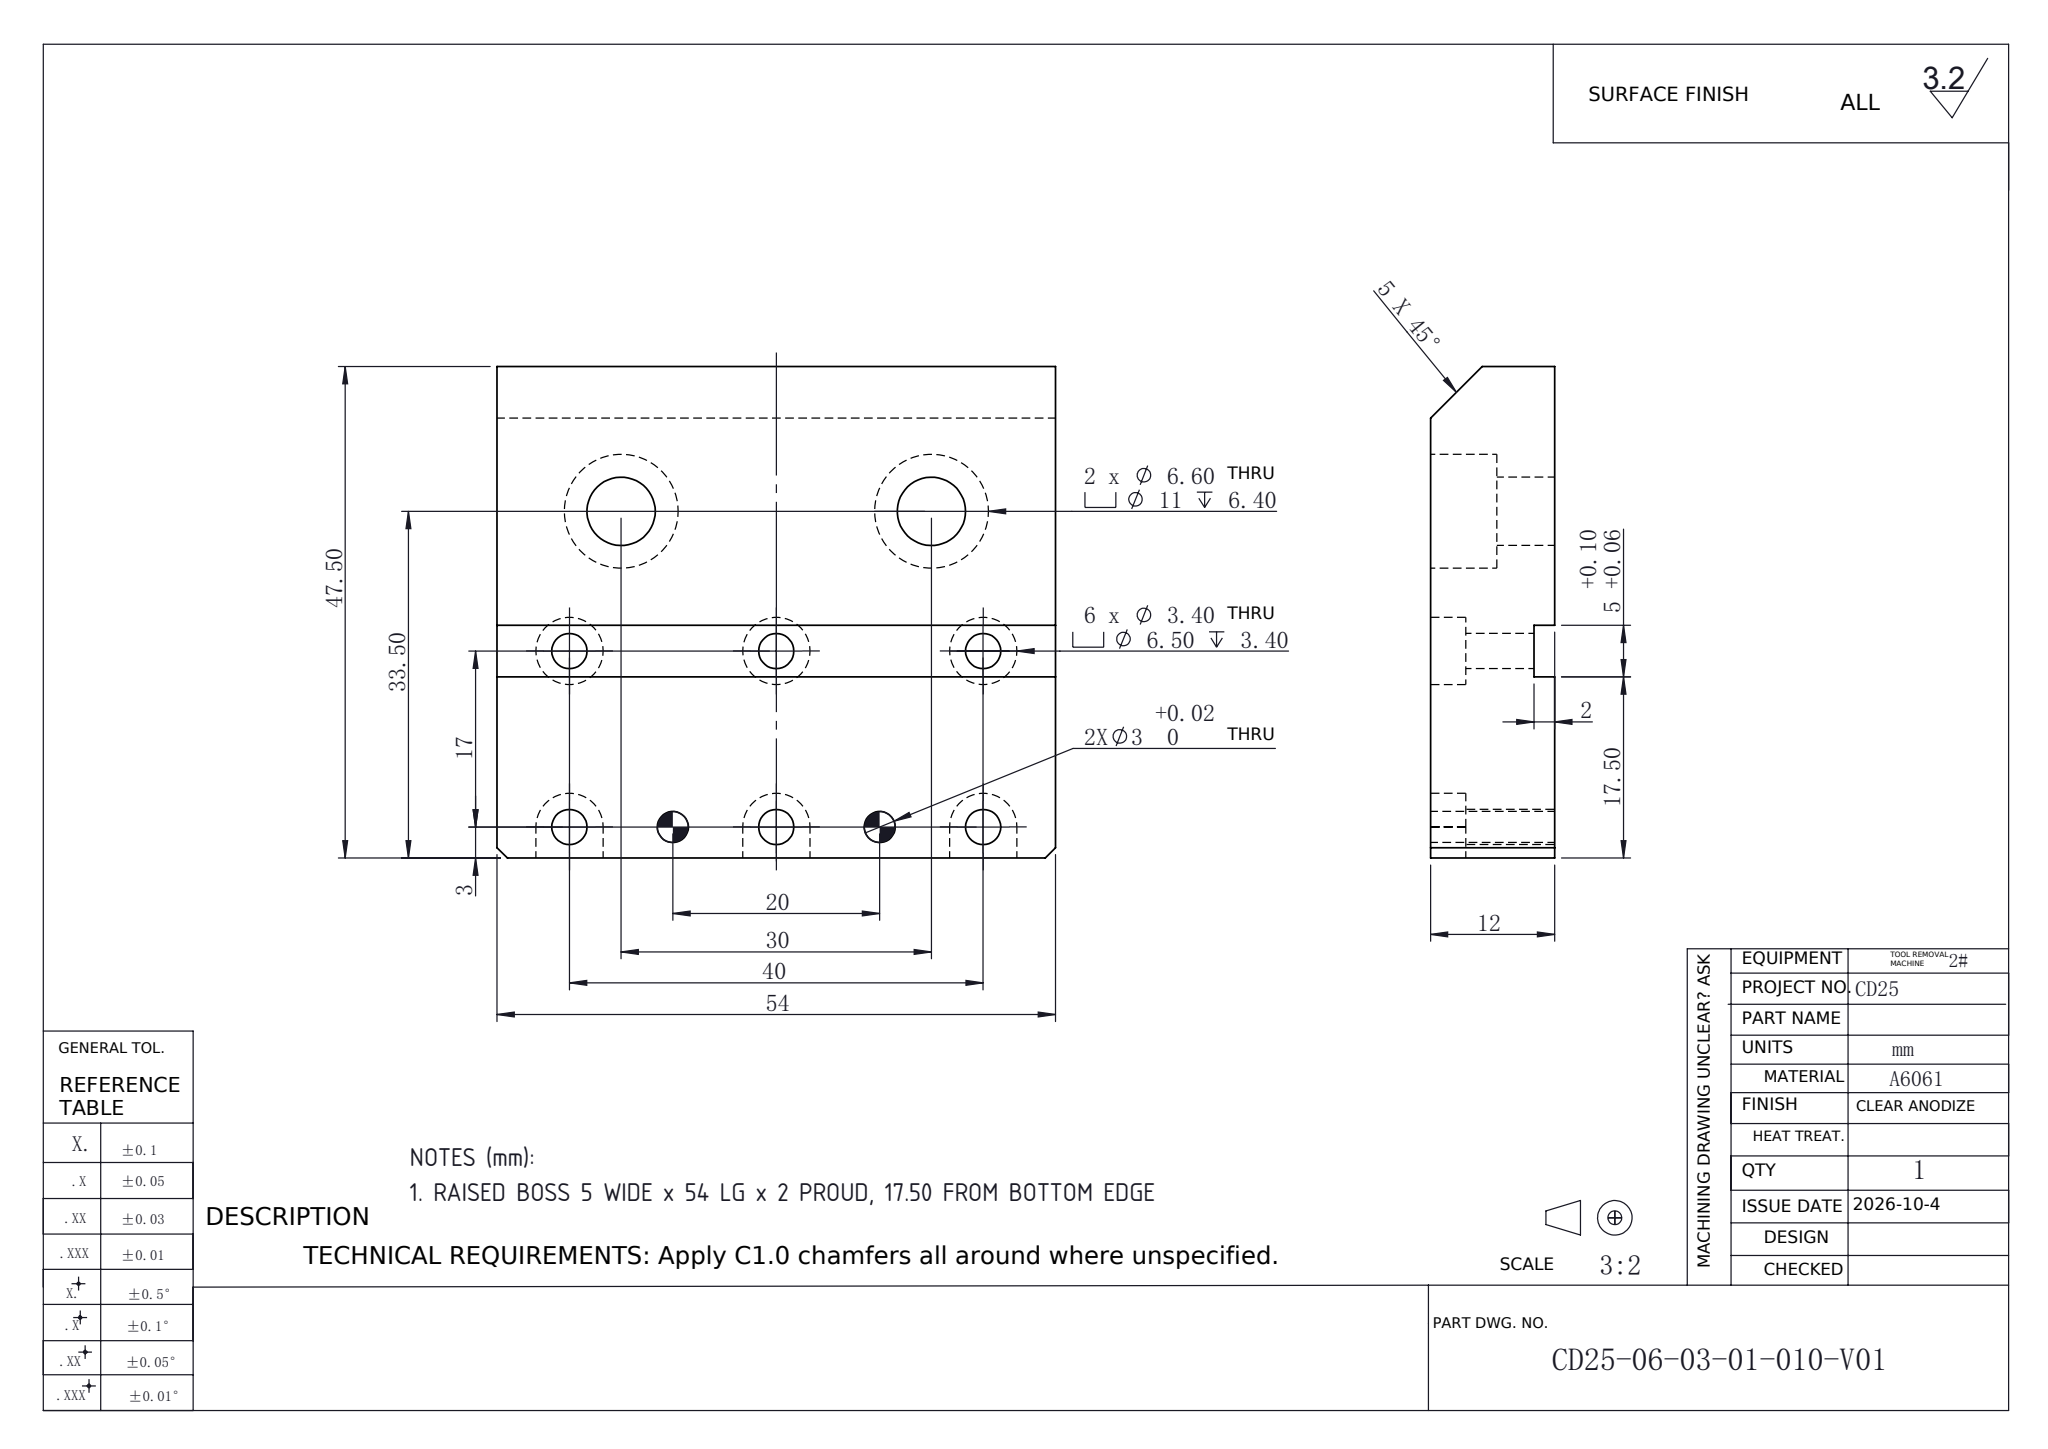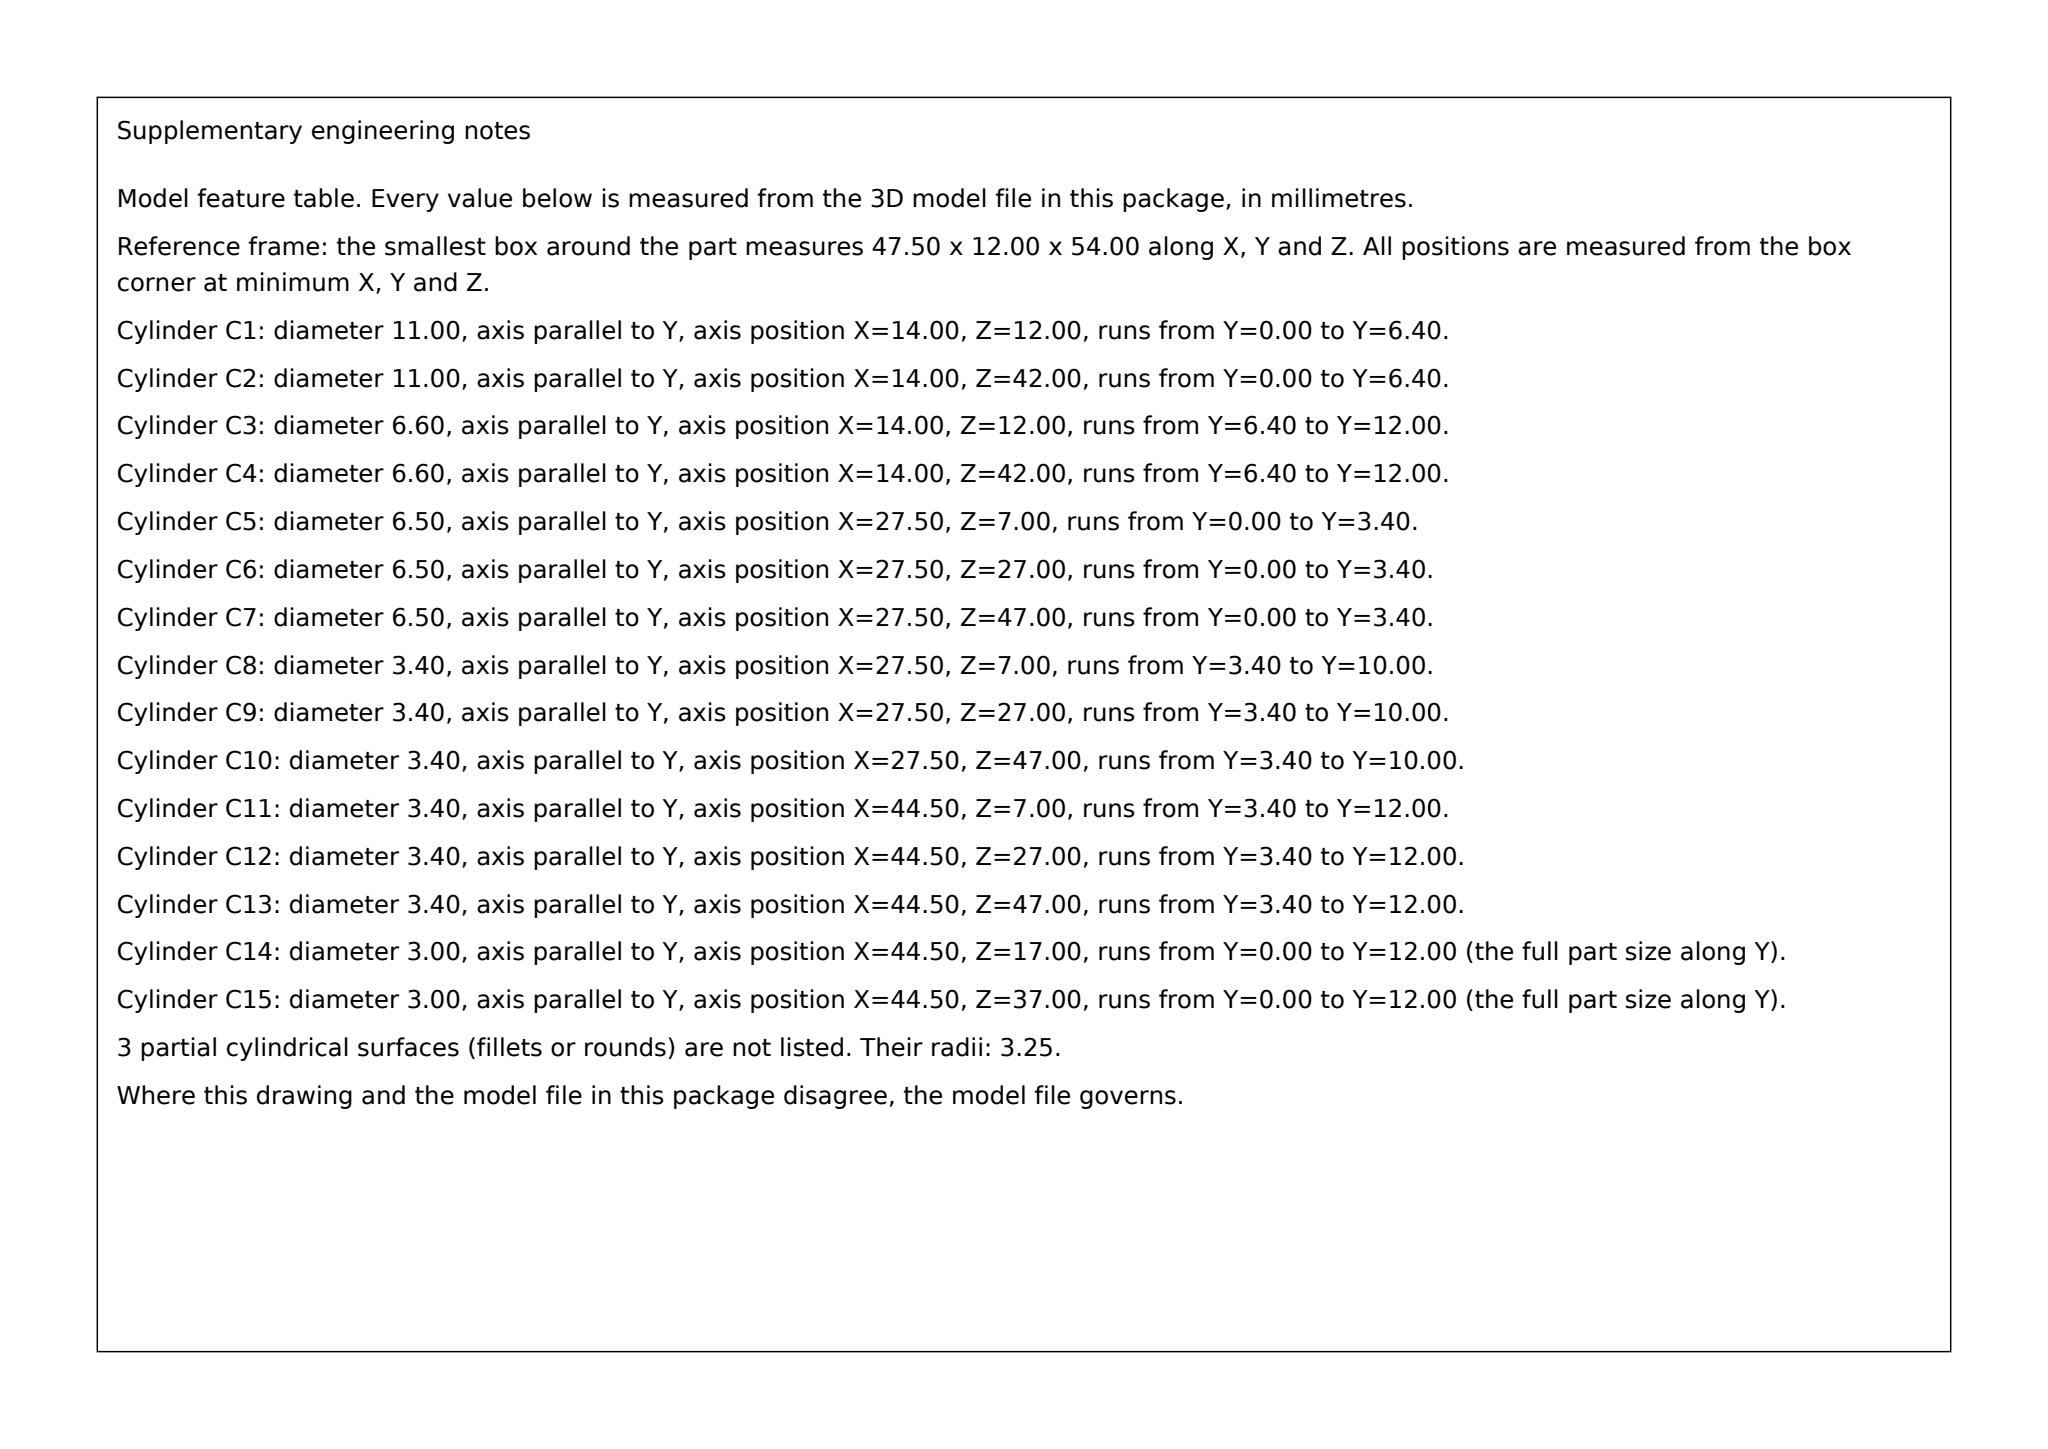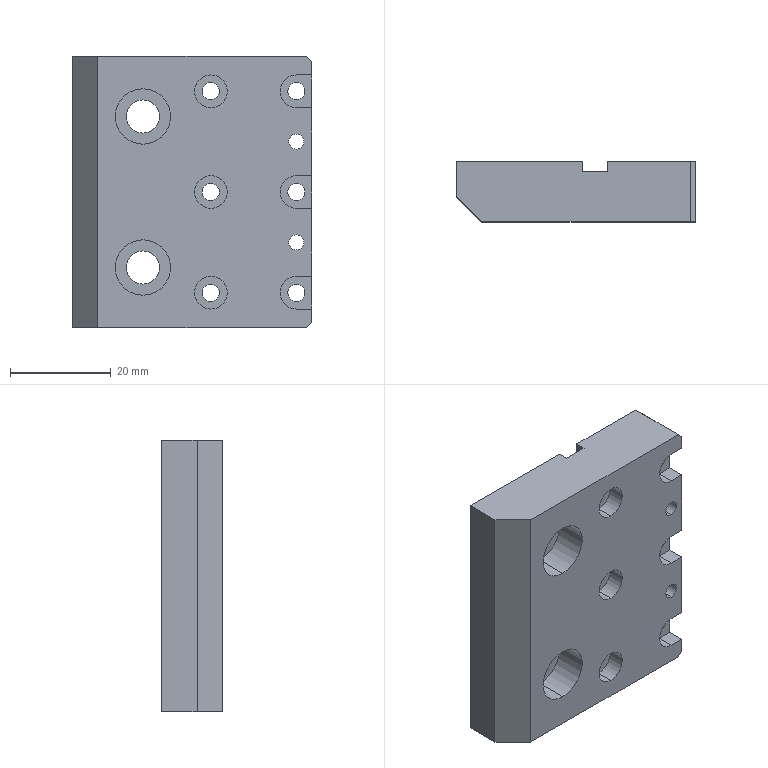Part | SolidWorks | mm | 1 solid | 60 faces | box 47.5 x 12 x 54 mm | volume 26663 mm3 | cylinder 33 | plane 27 | commonest cylinder face diameters 3.4 x12 6.5 x9 3 x4 11 x4 6.6 x4
Drawing notes:
RAISED BOSS 5 WIDE x 54 LG x 2 PROUD, 17.50 FROM BOTTOM EDGE | from the solid: x-planes at 25.0 & 30.0 (5 wide) on 47.5 height => 17.5 to 22.5 from bottom edge; boss spans full z=0 to 54; y-planes 10.0 to 12.0 give 2 thk
build123d program:
from build123d import *

# Parameters (mm, degrees)
SKETCH1_W                                       = 47.5
SKETCH1_H                                       = 54
BOSS_EXTRUDE1_DEPTH                             = 6
M6_HEX_SOCKET_HEAD_CAP_SCREW_CBORE1_D           = 6.6
M6_HEX_SOCKET_HEAD_CAP_SCREW_CBORE1_CBORE_D     = 11
M6_HEX_SOCKET_HEAD_CAP_SCREW_CBORE1_CBORE_DEPTH = 6.4
M3_HEX_SOCKET_HEAD_CAP_SCREW_CBORE1_D           = 3.4
M3_HEX_SOCKET_HEAD_CAP_SCREW_CBORE1_CBORE_D     = 6.5
M3_HEX_SOCKET_HEAD_CAP_SCREW_CBORE1_CBORE_DEPTH = 3.4
F_3_0MM_DOWEL_PIN_HOLE1_D                       = 3
CUT_EXTRUDE1_DEPTH                              = 3.4
CHAMFER1_SIZE                                   = 1
SKETCH10_W                                      = 5
SKETCH10_H                                      = 2
CUT_EXTRUDE2_DEPTH                              = 60.296
CHAMFER2_SIZE                                   = 5


with BuildPart() as part:
    # Sketch1 → Boss-Extrude1 (new, symmetric)
    with BuildSketch(Plane(origin=(0, 0, 0), x_dir=(1, 0, 0), z_dir=(0, 1, 0))):
        Rectangle(SKETCH1_W, SKETCH1_H)
    extrude(amount=BOSS_EXTRUDE1_DEPTH, both=True)

    # M6 Hex Socket Head Cap Screw CBORE1 (through all)
    with Locations(Plane(origin=(0, -6, 0), x_dir=(-1, 0, 0), z_dir=(0, -1, 0))):
        with Locations((9.75, 15), (9.75, -15)):
            CounterBoreHole(M6_HEX_SOCKET_HEAD_CAP_SCREW_CBORE1_D / 2, M6_HEX_SOCKET_HEAD_CAP_SCREW_CBORE1_CBORE_D / 2, M6_HEX_SOCKET_HEAD_CAP_SCREW_CBORE1_CBORE_DEPTH)

    # M3 Hex Socket Head Cap Screw CBORE1 (through all)
    with Locations(Plane(origin=(0, -6, 0), x_dir=(-1, 0, 0), z_dir=(0, -1, 0))):
        with Locations((-20.75, -20), (-20.75, 0), (-20.75, 20), (-3.75, 20), (-3.75, 0), (-3.75, -20)):
            CounterBoreHole(M3_HEX_SOCKET_HEAD_CAP_SCREW_CBORE1_D / 2, M3_HEX_SOCKET_HEAD_CAP_SCREW_CBORE1_CBORE_D / 2, M3_HEX_SOCKET_HEAD_CAP_SCREW_CBORE1_CBORE_DEPTH)

    # 3.0mm Dowel Pin Hole1 (through all)
    with Locations(Plane(origin=(0, -6, 0), x_dir=(-1, 0, 0), z_dir=(0, -1, 0))):
        with Locations((-20.75, 10), (-20.75, -10)):
            Hole(F_3_0MM_DOWEL_PIN_HOLE1_D / 2)

    # Sketch9 → Cut-Extrude1 (cut)
    with BuildSketch(Plane.XZ.offset(6)):
        with BuildLine():
            Line((20.75, 23.25), (23.75, 23.25))
            ThreePointArc((23.75, 23.25), (27, 20), (23.75, 16.75))
            Line((23.75, 16.75), (20.75, 16.75))
            ThreePointArc((20.75, 16.75), (17.5, 20), (20.75, 23.25))
        make_face()
        with BuildLine():
            Line((20.75, -23.25), (23.75, -23.25))
            ThreePointArc((23.75, -23.25), (27, -20), (23.75, -16.75))
            Line((23.75, -16.75), (20.75, -16.75))
            ThreePointArc((20.75, -16.75), (17.5, -20), (20.75, -23.25))
        make_face()
        with BuildLine():
            Line((20.75, 3.25), (23.75, 3.25))
            ThreePointArc((23.75, 3.25), (27, 0), (23.75, -3.25))
            Line((23.75, -3.25), (20.75, -3.25))
            ThreePointArc((20.75, -3.25), (17.5, 0), (20.75, 3.25))
        make_face()
    extrude(amount=-CUT_EXTRUDE1_DEPTH, mode=Mode.SUBTRACT)

    # Chamfer1
    chamfer1_edges = [part.edges().sort_by_distance(p)[0] for p in [
        (23.75, 0, 27),
        (23.75, 0, -27),
    ]]
    chamfer(chamfer1_edges, length=CHAMFER1_SIZE)

    # Sketch10 → Cut-Extrude2 (cut, through all)
    with BuildSketch(Plane(origin=(0, 0, -27), x_dir=(-1, 0, 0), z_dir=(0, 0, -1))):
        with Locations((-3.75, 5)):
            Rectangle(SKETCH10_W, SKETCH10_H)
    extrude(amount=-CUT_EXTRUDE2_DEPTH, mode=Mode.SUBTRACT)

    # Chamfer2
    chamfer2_edges = [part.edges().sort_by_distance(p)[0] for p in [
        (-23.75, -6, 0),
    ]]
    chamfer(chamfer2_edges, length=CHAMFER2_SIZE)


solid = part.part